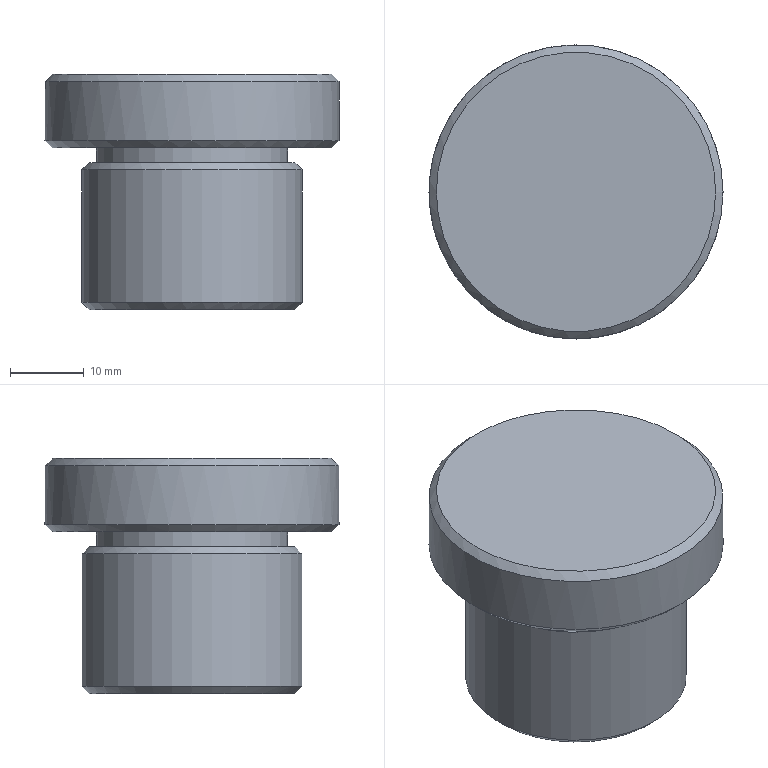Component | NX | DOWEL_PIN | 1 solid | 11 faces | box 40 x 40 x 32 mm | volume 27550 mm3 | plane 4 | cone 4 | cylinder 3 | commonest cylinder face diameters 30 x1 26 x1 40 x1
STEP:
#1=CARTESIAN_POINT('',(0.,0.,0.));
#2=DIRECTION('',(0.,0.,1.));
#3=DIRECTION('',(1.,0.,0.));
#4=AXIS2_PLACEMENT_3D('',#1,#2,#3);
#5=CARTESIAN_POINT('',(14.,0.,71.));
#6=VERTEX_POINT('',#5);
#7=CARTESIAN_POINT('',(0.,0.,71.));
#8=DIRECTION('',(0.,0.,1.));
#9=DIRECTION('',(1.,0.,0.));
#10=AXIS2_PLACEMENT_3D('',#7,#8,#9);
#11=CIRCLE('',#10,14.);
#12=CARTESIAN_POINT('',(0.,0.,71.));
#13=DIRECTION('',(0.,0.,1.));
#14=DIRECTION('',(1.,0.,0.));
#15=AXIS2_PLACEMENT_3D('',#12,#13,#14);
#16=PLANE('',#15);
#17=CARTESIAN_POINT('',(0.,0.));
#18=DIRECTION('',(1.,0.));
#19=AXIS2_PLACEMENT_2D('',#17,#18);
#20=CIRCLE('',#19,14.);
#21=(GEOMETRIC_REPRESENTATION_CONTEXT(2)PARAMETRIC_REPRESENTATION_CONTEXT()REPRESENTATION_CONTEXT('',''));
#22=DEFINITIONAL_REPRESENTATION('',(#20),#21);
#23=PCURVE('',#16,#22);
#24=CARTESIAN_POINT('',(0.,0.,70.));
#25=DIRECTION('',(0.,0.,-1.));
#26=DIRECTION('',(-1.,0.,0.));
#27=AXIS2_PLACEMENT_3D('',#24,#25,#26);
#28=CONICAL_SURFACE('',#27,15.,0.7854);
#29=CARTESIAN_POINT('',(9.425,-1.));
#30=DIRECTION('',(-1.,0.));
#31=VECTOR('',#30,1.);
#32=LINE('',#29,#31);
#33=(GEOMETRIC_REPRESENTATION_CONTEXT(2)PARAMETRIC_REPRESENTATION_CONTEXT()REPRESENTATION_CONTEXT('',''));
#34=DEFINITIONAL_REPRESENTATION('',(#32),#33);
#35=PCURVE('',#28,#34);
#36=SURFACE_CURVE('',#11,(#23,#35),.PCURVE_S1.);
#37=EDGE_CURVE('',#6,#6,#36,.T.);
#38=ORIENTED_EDGE('',*,*,#37,.T.);
#39=EDGE_LOOP('',(#38));
#40=FACE_BOUND('',#39,.T.);
#41=CARTESIAN_POINT('',(13.,0.,71.));
#42=VERTEX_POINT('',#41);
#43=CARTESIAN_POINT('',(0.,0.,71.));
#44=DIRECTION('',(0.,0.,1.));
#45=DIRECTION('',(1.,0.,0.));
#46=AXIS2_PLACEMENT_3D('',#43,#44,#45);
#47=CIRCLE('',#46,13.);
#48=CARTESIAN_POINT('',(0.,0.));
#49=DIRECTION('',(1.,0.));
#50=AXIS2_PLACEMENT_2D('',#48,#49);
#51=CIRCLE('',#50,13.);
#52=(GEOMETRIC_REPRESENTATION_CONTEXT(2)PARAMETRIC_REPRESENTATION_CONTEXT()REPRESENTATION_CONTEXT('',''));
#53=DEFINITIONAL_REPRESENTATION('',(#51),#52);
#54=PCURVE('',#16,#53);
#55=CARTESIAN_POINT('',(0.,0.,71.));
#56=DIRECTION('',(0.,0.,1.));
#57=DIRECTION('',(1.,0.,0.));
#58=AXIS2_PLACEMENT_3D('',#55,#56,#57);
#59=CYLINDRICAL_SURFACE('',#58,13.);
#60=CARTESIAN_POINT('',(0.,0.));
#61=DIRECTION('',(1.,0.));
#62=VECTOR('',#61,1.);
#63=LINE('',#60,#62);
#64=(GEOMETRIC_REPRESENTATION_CONTEXT(2)PARAMETRIC_REPRESENTATION_CONTEXT()REPRESENTATION_CONTEXT('',''));
#65=DEFINITIONAL_REPRESENTATION('',(#63),#64);
#66=PCURVE('',#59,#65);
#67=SURFACE_CURVE('',#47,(#54,#66),.PCURVE_S1.);
#68=EDGE_CURVE('',#42,#42,#67,.T.);
#69=ORIENTED_EDGE('',*,*,#68,.F.);
#70=EDGE_LOOP('',(#69));
#71=FACE_BOUND('',#70,.T.);
#72=ADVANCED_FACE('',(#40,#71),#16,.T.);
#73=CARTESIAN_POINT('',(-14.,0.,51.));
#74=VERTEX_POINT('',#73);
#75=CARTESIAN_POINT('',(0.,0.,51.));
#76=DIRECTION('',(0.,0.,-1.));
#77=DIRECTION('',(-1.,0.,0.));
#78=AXIS2_PLACEMENT_3D('',#75,#76,#77);
#79=CIRCLE('',#78,14.);
#80=CARTESIAN_POINT('',(0.,0.,51.));
#81=DIRECTION('',(0.,0.,-1.));
#82=DIRECTION('',(-1.,0.,0.));
#83=AXIS2_PLACEMENT_3D('',#80,#81,#82);
#84=PLANE('',#83);
#85=CARTESIAN_POINT('',(0.,0.));
#86=DIRECTION('',(1.,0.));
#87=AXIS2_PLACEMENT_2D('',#85,#86);
#88=CIRCLE('',#87,14.);
#89=(GEOMETRIC_REPRESENTATION_CONTEXT(2)PARAMETRIC_REPRESENTATION_CONTEXT()REPRESENTATION_CONTEXT('',''));
#90=DEFINITIONAL_REPRESENTATION('',(#88),#89);
#91=PCURVE('',#84,#90);
#92=CARTESIAN_POINT('',(0.,0.,52.));
#93=DIRECTION('',(0.,0.,1.));
#94=DIRECTION('',(1.,0.,0.));
#95=AXIS2_PLACEMENT_3D('',#92,#93,#94);
#96=CONICAL_SURFACE('',#95,15.,0.7854);
#97=CARTESIAN_POINT('',(9.425,-1.));
#98=DIRECTION('',(-1.,0.));
#99=VECTOR('',#98,1.);
#100=LINE('',#97,#99);
#101=(GEOMETRIC_REPRESENTATION_CONTEXT(2)PARAMETRIC_REPRESENTATION_CONTEXT()REPRESENTATION_CONTEXT('',''));
#102=DEFINITIONAL_REPRESENTATION('',(#100),#101);
#103=PCURVE('',#96,#102);
#104=SURFACE_CURVE('',#79,(#91,#103),.PCURVE_S1.);
#105=EDGE_CURVE('',#74,#74,#104,.T.);
#106=ORIENTED_EDGE('',*,*,#105,.T.);
#107=EDGE_LOOP('',(#106));
#108=FACE_BOUND('',#107,.T.);
#109=ADVANCED_FACE('',(#108),#84,.T.);
#110=CARTESIAN_POINT('',(-15.,0.,52.));
#111=VERTEX_POINT('',#110);
#112=CARTESIAN_POINT('',(15.,-0.,52.));
#113=VERTEX_POINT('',#112);
#114=CARTESIAN_POINT('',(0.,0.,52.));
#115=DIRECTION('',(0.,0.,1.));
#116=DIRECTION('',(-1.,0.,0.));
#117=AXIS2_PLACEMENT_3D('',#114,#115,#116);
#118=CIRCLE('',#117,15.);
#119=CARTESIAN_POINT('',(0.,0.,51.));
#120=DIRECTION('',(0.,0.,1.));
#121=DIRECTION('',(1.,0.,0.));
#122=AXIS2_PLACEMENT_3D('',#119,#120,#121);
#123=CYLINDRICAL_SURFACE('',#122,15.);
#124=CARTESIAN_POINT('',(3.142,1.));
#125=DIRECTION('',(1.,0.));
#126=VECTOR('',#125,1.);
#127=LINE('',#124,#126);
#128=(GEOMETRIC_REPRESENTATION_CONTEXT(2)PARAMETRIC_REPRESENTATION_CONTEXT()REPRESENTATION_CONTEXT('',''));
#129=DEFINITIONAL_REPRESENTATION('',(#127),#128);
#130=PCURVE('',#123,#129);
#131=CARTESIAN_POINT('',(3.142,0.));
#132=DIRECTION('',(1.,0.));
#133=VECTOR('',#132,1.);
#134=LINE('',#131,#133);
#135=(GEOMETRIC_REPRESENTATION_CONTEXT(2)PARAMETRIC_REPRESENTATION_CONTEXT()REPRESENTATION_CONTEXT('',''));
#136=DEFINITIONAL_REPRESENTATION('',(#134),#135);
#137=PCURVE('',#96,#136);
#138=SURFACE_CURVE('',#118,(#130,#137),.PCURVE_S1.);
#139=EDGE_CURVE('',#111,#113,#138,.T.);
#140=ORIENTED_EDGE('',*,*,#139,.T.);
#141=CARTESIAN_POINT('',(15.,0.,70.));
#142=VERTEX_POINT('',#141);
#143=CARTESIAN_POINT('',(15.,0.,52.));
#144=CARTESIAN_POINT('',(15.,0.,70.));
#145=B_SPLINE_CURVE_WITH_KNOTS('',1,(#143,#144),.UNSPECIFIED.,.F.,.F.,(2,2),(1.,19.),.PIECEWISE_BEZIER_KNOTS.);
#146=CARTESIAN_POINT('',(6.283,0.));
#147=DIRECTION('',(0.,1.));
#148=VECTOR('',#147,1.);
#149=LINE('',#146,#148);
#150=(GEOMETRIC_REPRESENTATION_CONTEXT(2)PARAMETRIC_REPRESENTATION_CONTEXT()REPRESENTATION_CONTEXT('',''));
#151=DEFINITIONAL_REPRESENTATION('',(#149),#150);
#152=PCURVE('',#123,#151);
#153=CARTESIAN_POINT('',(0.,0.));
#154=DIRECTION('',(0.,1.));
#155=VECTOR('',#154,1.);
#156=LINE('',#153,#155);
#157=(GEOMETRIC_REPRESENTATION_CONTEXT(2)PARAMETRIC_REPRESENTATION_CONTEXT()REPRESENTATION_CONTEXT('',''));
#158=DEFINITIONAL_REPRESENTATION('',(#156),#157);
#159=PCURVE('',#123,#158);
#160=SEAM_CURVE('',#145,(#152,#159),.PCURVE_S1.);
#161=EDGE_CURVE('',#113,#142,#160,.T.);
#162=ORIENTED_EDGE('',*,*,#161,.T.);
#163=CARTESIAN_POINT('',(0.,0.,70.));
#164=DIRECTION('',(0.,0.,-1.));
#165=DIRECTION('',(1.,0.,0.));
#166=AXIS2_PLACEMENT_3D('',#163,#164,#165);
#167=CIRCLE('',#166,15.);
#168=CARTESIAN_POINT('',(6.283,19.));
#169=DIRECTION('',(-1.,0.));
#170=VECTOR('',#169,1.);
#171=LINE('',#168,#170);
#172=(GEOMETRIC_REPRESENTATION_CONTEXT(2)PARAMETRIC_REPRESENTATION_CONTEXT()REPRESENTATION_CONTEXT('',''));
#173=DEFINITIONAL_REPRESENTATION('',(#171),#172);
#174=PCURVE('',#123,#173);
#175=CARTESIAN_POINT('',(3.142,0.));
#176=DIRECTION('',(1.,0.));
#177=VECTOR('',#176,1.);
#178=LINE('',#175,#177);
#179=(GEOMETRIC_REPRESENTATION_CONTEXT(2)PARAMETRIC_REPRESENTATION_CONTEXT()REPRESENTATION_CONTEXT('',''));
#180=DEFINITIONAL_REPRESENTATION('',(#178),#179);
#181=PCURVE('',#28,#180);
#182=SURFACE_CURVE('',#167,(#174,#181),.PCURVE_S1.);
#183=EDGE_CURVE('',#142,#142,#182,.T.);
#184=ORIENTED_EDGE('',*,*,#183,.T.);
#185=ORIENTED_EDGE('',*,*,#161,.F.);
#186=CARTESIAN_POINT('',(0.,0.,52.));
#187=DIRECTION('',(0.,0.,1.));
#188=DIRECTION('',(-1.,0.,0.));
#189=AXIS2_PLACEMENT_3D('',#186,#187,#188);
#190=CIRCLE('',#189,15.);
#191=CARTESIAN_POINT('',(-3.142,1.));
#192=DIRECTION('',(1.,0.));
#193=VECTOR('',#192,1.);
#194=LINE('',#191,#193);
#195=(GEOMETRIC_REPRESENTATION_CONTEXT(2)PARAMETRIC_REPRESENTATION_CONTEXT()REPRESENTATION_CONTEXT('',''));
#196=DEFINITIONAL_REPRESENTATION('',(#194),#195);
#197=PCURVE('',#123,#196);
#198=CARTESIAN_POINT('',(3.142,0.));
#199=DIRECTION('',(1.,0.));
#200=VECTOR('',#199,1.);
#201=LINE('',#198,#200);
#202=(GEOMETRIC_REPRESENTATION_CONTEXT(2)PARAMETRIC_REPRESENTATION_CONTEXT()REPRESENTATION_CONTEXT('',''));
#203=DEFINITIONAL_REPRESENTATION('',(#201),#202);
#204=PCURVE('',#96,#203);
#205=SURFACE_CURVE('',#190,(#197,#204),.PCURVE_S1.);
#206=EDGE_CURVE('',#113,#111,#205,.T.);
#207=ORIENTED_EDGE('',*,*,#206,.T.);
#208=EDGE_LOOP('',(#140,#162,#184,#185,#207));
#209=FACE_BOUND('',#208,.T.);
#210=ADVANCED_FACE('',(#209),#123,.T.);
#211=CARTESIAN_POINT('',(13.,0.,73.));
#212=VERTEX_POINT('',#211);
#213=CARTESIAN_POINT('',(-13.,0.,73.));
#214=VERTEX_POINT('',#213);
#215=CARTESIAN_POINT('',(0.,0.,73.));
#216=DIRECTION('',(0.,0.,1.));
#217=DIRECTION('',(-1.,0.,0.));
#218=AXIS2_PLACEMENT_3D('',#215,#216,#217);
#219=CIRCLE('',#218,13.);
#220=CARTESIAN_POINT('',(-3.142,2.));
#221=DIRECTION('',(1.,0.));
#222=VECTOR('',#221,1.);
#223=LINE('',#220,#222);
#224=(GEOMETRIC_REPRESENTATION_CONTEXT(2)PARAMETRIC_REPRESENTATION_CONTEXT()REPRESENTATION_CONTEXT('',''));
#225=DEFINITIONAL_REPRESENTATION('',(#223),#224);
#226=PCURVE('',#59,#225);
#227=CARTESIAN_POINT('',(0.,0.,73.));
#228=DIRECTION('',(0.,0.,-1.));
#229=DIRECTION('',(-1.,0.,0.));
#230=AXIS2_PLACEMENT_3D('',#227,#228,#229);
#231=PLANE('',#230);
#232=CARTESIAN_POINT('',(13.,0.));
#233=CARTESIAN_POINT('',(13.,-22.517));
#234=CARTESIAN_POINT('',(-6.5,-11.258));
#235=CARTESIAN_POINT('',(-26.,-0.));
#236=CARTESIAN_POINT('',(-6.5,11.258));
#237=CARTESIAN_POINT('',(13.,22.517));
#238=CARTESIAN_POINT('',(13.,0.));
#239=(BOUNDED_CURVE()B_SPLINE_CURVE(2,(#232,#233,#234,#235,#236,#237,#238),.UNSPECIFIED.,.T.,.F.)B_SPLINE_CURVE_WITH_KNOTS((1,2,2,2,2,1),(-2.094,0.,2.094,4.189,6.283,8.378),.UNSPECIFIED.)CURVE()GEOMETRIC_REPRESENTATION_ITEM()RATIONAL_B_SPLINE_CURVE((1.,0.5,1.,0.5,1.,0.5,1.))REPRESENTATION_ITEM(''));
#240=(GEOMETRIC_REPRESENTATION_CONTEXT(2)PARAMETRIC_REPRESENTATION_CONTEXT()REPRESENTATION_CONTEXT('',''));
#241=DEFINITIONAL_REPRESENTATION('',(#239),#240);
#242=PCURVE('',#231,#241);
#243=SURFACE_CURVE('',#219,(#226,#242),.PCURVE_S1.);
#244=EDGE_CURVE('',#212,#214,#243,.T.);
#245=ORIENTED_EDGE('',*,*,#244,.F.);
#246=CARTESIAN_POINT('',(13.,-0.,71.));
#247=CARTESIAN_POINT('',(13.,-0.,73.));
#248=B_SPLINE_CURVE_WITH_KNOTS('',1,(#246,#247),.UNSPECIFIED.,.F.,.F.,(2,2),(0.,2.),.PIECEWISE_BEZIER_KNOTS.);
#249=CARTESIAN_POINT('',(0.,0.));
#250=DIRECTION('',(0.,1.));
#251=VECTOR('',#250,1.);
#252=LINE('',#249,#251);
#253=(GEOMETRIC_REPRESENTATION_CONTEXT(2)PARAMETRIC_REPRESENTATION_CONTEXT()REPRESENTATION_CONTEXT('',''));
#254=DEFINITIONAL_REPRESENTATION('',(#252),#253);
#255=PCURVE('',#59,#254);
#256=CARTESIAN_POINT('',(6.283,0.));
#257=DIRECTION('',(0.,1.));
#258=VECTOR('',#257,1.);
#259=LINE('',#256,#258);
#260=(GEOMETRIC_REPRESENTATION_CONTEXT(2)PARAMETRIC_REPRESENTATION_CONTEXT()REPRESENTATION_CONTEXT('',''));
#261=DEFINITIONAL_REPRESENTATION('',(#259),#260);
#262=PCURVE('',#59,#261);
#263=SEAM_CURVE('',#248,(#255,#262),.PCURVE_S1.);
#264=EDGE_CURVE('',#42,#212,#263,.T.);
#265=ORIENTED_EDGE('',*,*,#264,.F.);
#266=ORIENTED_EDGE('',*,*,#68,.T.);
#267=ORIENTED_EDGE('',*,*,#264,.T.);
#268=CARTESIAN_POINT('',(0.,0.,73.));
#269=DIRECTION('',(0.,0.,1.));
#270=DIRECTION('',(-1.,0.,0.));
#271=AXIS2_PLACEMENT_3D('',#268,#269,#270);
#272=CIRCLE('',#271,13.);
#273=CARTESIAN_POINT('',(3.142,2.));
#274=DIRECTION('',(1.,0.));
#275=VECTOR('',#274,1.);
#276=LINE('',#273,#275);
#277=(GEOMETRIC_REPRESENTATION_CONTEXT(2)PARAMETRIC_REPRESENTATION_CONTEXT()REPRESENTATION_CONTEXT('',''));
#278=DEFINITIONAL_REPRESENTATION('',(#276),#277);
#279=PCURVE('',#59,#278);
#280=CARTESIAN_POINT('',(13.,0.));
#281=CARTESIAN_POINT('',(13.,-22.517));
#282=CARTESIAN_POINT('',(-6.5,-11.258));
#283=CARTESIAN_POINT('',(-26.,-0.));
#284=CARTESIAN_POINT('',(-6.5,11.258));
#285=CARTESIAN_POINT('',(13.,22.517));
#286=CARTESIAN_POINT('',(13.,0.));
#287=(BOUNDED_CURVE()B_SPLINE_CURVE(2,(#280,#281,#282,#283,#284,#285,#286),.UNSPECIFIED.,.T.,.F.)B_SPLINE_CURVE_WITH_KNOTS((1,2,2,2,2,1),(-2.094,0.,2.094,4.189,6.283,8.378),.UNSPECIFIED.)CURVE()GEOMETRIC_REPRESENTATION_ITEM()RATIONAL_B_SPLINE_CURVE((1.,0.5,1.,0.5,1.,0.5,1.))REPRESENTATION_ITEM(''));
#288=(GEOMETRIC_REPRESENTATION_CONTEXT(2)PARAMETRIC_REPRESENTATION_CONTEXT()REPRESENTATION_CONTEXT('',''));
#289=DEFINITIONAL_REPRESENTATION('',(#287),#288);
#290=PCURVE('',#231,#289);
#291=SURFACE_CURVE('',#272,(#279,#290),.PCURVE_S1.);
#292=EDGE_CURVE('',#214,#212,#291,.T.);
#293=ORIENTED_EDGE('',*,*,#292,.F.);
#294=EDGE_LOOP('',(#245,#265,#266,#267,#293));
#295=FACE_BOUND('',#294,.T.);
#296=ADVANCED_FACE('',(#295),#59,.T.);
#297=CARTESIAN_POINT('',(19.,0.,83.));
#298=VERTEX_POINT('',#297);
#299=CARTESIAN_POINT('',(0.,0.,83.));
#300=DIRECTION('',(0.,0.,1.));
#301=DIRECTION('',(1.,0.,0.));
#302=AXIS2_PLACEMENT_3D('',#299,#300,#301);
#303=CIRCLE('',#302,19.);
#304=CARTESIAN_POINT('',(0.,0.,83.));
#305=DIRECTION('',(0.,0.,1.));
#306=DIRECTION('',(1.,0.,0.));
#307=AXIS2_PLACEMENT_3D('',#304,#305,#306);
#308=PLANE('',#307);
#309=CARTESIAN_POINT('',(0.,0.));
#310=DIRECTION('',(1.,0.));
#311=AXIS2_PLACEMENT_2D('',#309,#310);
#312=CIRCLE('',#311,19.);
#313=(GEOMETRIC_REPRESENTATION_CONTEXT(2)PARAMETRIC_REPRESENTATION_CONTEXT()REPRESENTATION_CONTEXT('',''));
#314=DEFINITIONAL_REPRESENTATION('',(#312),#313);
#315=PCURVE('',#308,#314);
#316=CARTESIAN_POINT('',(0.,0.,82.));
#317=DIRECTION('',(0.,0.,-1.));
#318=DIRECTION('',(-1.,0.,0.));
#319=AXIS2_PLACEMENT_3D('',#316,#317,#318);
#320=CONICAL_SURFACE('',#319,20.,0.7854);
#321=CARTESIAN_POINT('',(9.425,-1.));
#322=DIRECTION('',(-1.,0.));
#323=VECTOR('',#322,1.);
#324=LINE('',#321,#323);
#325=(GEOMETRIC_REPRESENTATION_CONTEXT(2)PARAMETRIC_REPRESENTATION_CONTEXT()REPRESENTATION_CONTEXT('',''));
#326=DEFINITIONAL_REPRESENTATION('',(#324),#325);
#327=PCURVE('',#320,#326);
#328=SURFACE_CURVE('',#303,(#315,#327),.PCURVE_S1.);
#329=EDGE_CURVE('',#298,#298,#328,.T.);
#330=ORIENTED_EDGE('',*,*,#329,.T.);
#331=EDGE_LOOP('',(#330));
#332=FACE_BOUND('',#331,.T.);
#333=ADVANCED_FACE('',(#332),#308,.T.);
#334=CARTESIAN_POINT('',(-19.,0.,73.));
#335=VERTEX_POINT('',#334);
#336=CARTESIAN_POINT('',(0.,0.,73.));
#337=DIRECTION('',(0.,0.,-1.));
#338=DIRECTION('',(-1.,0.,0.));
#339=AXIS2_PLACEMENT_3D('',#336,#337,#338);
#340=CIRCLE('',#339,19.);
#341=CARTESIAN_POINT('',(0.,0.));
#342=DIRECTION('',(1.,0.));
#343=AXIS2_PLACEMENT_2D('',#341,#342);
#344=CIRCLE('',#343,19.);
#345=(GEOMETRIC_REPRESENTATION_CONTEXT(2)PARAMETRIC_REPRESENTATION_CONTEXT()REPRESENTATION_CONTEXT('',''));
#346=DEFINITIONAL_REPRESENTATION('',(#344),#345);
#347=PCURVE('',#231,#346);
#348=CARTESIAN_POINT('',(0.,0.,74.));
#349=DIRECTION('',(0.,0.,1.));
#350=DIRECTION('',(1.,0.,0.));
#351=AXIS2_PLACEMENT_3D('',#348,#349,#350);
#352=CONICAL_SURFACE('',#351,20.,0.7854);
#353=CARTESIAN_POINT('',(9.425,-1.));
#354=DIRECTION('',(-1.,0.));
#355=VECTOR('',#354,1.);
#356=LINE('',#353,#355);
#357=(GEOMETRIC_REPRESENTATION_CONTEXT(2)PARAMETRIC_REPRESENTATION_CONTEXT()REPRESENTATION_CONTEXT('',''));
#358=DEFINITIONAL_REPRESENTATION('',(#356),#357);
#359=PCURVE('',#352,#358);
#360=SURFACE_CURVE('',#340,(#347,#359),.PCURVE_S1.);
#361=EDGE_CURVE('',#335,#335,#360,.T.);
#362=ORIENTED_EDGE('',*,*,#361,.T.);
#363=EDGE_LOOP('',(#362));
#364=FACE_BOUND('',#363,.T.);
#365=ORIENTED_EDGE('',*,*,#292,.T.);
#366=ORIENTED_EDGE('',*,*,#244,.T.);
#367=EDGE_LOOP('',(#365,#366));
#368=FACE_BOUND('',#367,.T.);
#369=ADVANCED_FACE('',(#364,#368),#231,.T.);
#370=CARTESIAN_POINT('',(-20.,0.,74.));
#371=VERTEX_POINT('',#370);
#372=CARTESIAN_POINT('',(20.,-0.,74.));
#373=VERTEX_POINT('',#372);
#374=CARTESIAN_POINT('',(0.,0.,74.));
#375=DIRECTION('',(0.,0.,1.));
#376=DIRECTION('',(-1.,0.,0.));
#377=AXIS2_PLACEMENT_3D('',#374,#375,#376);
#378=CIRCLE('',#377,20.);
#379=CARTESIAN_POINT('',(0.,0.,73.));
#380=DIRECTION('',(0.,0.,1.));
#381=DIRECTION('',(1.,0.,0.));
#382=AXIS2_PLACEMENT_3D('',#379,#380,#381);
#383=CYLINDRICAL_SURFACE('',#382,20.);
#384=CARTESIAN_POINT('',(3.142,1.));
#385=DIRECTION('',(1.,0.));
#386=VECTOR('',#385,1.);
#387=LINE('',#384,#386);
#388=(GEOMETRIC_REPRESENTATION_CONTEXT(2)PARAMETRIC_REPRESENTATION_CONTEXT()REPRESENTATION_CONTEXT('',''));
#389=DEFINITIONAL_REPRESENTATION('',(#387),#388);
#390=PCURVE('',#383,#389);
#391=CARTESIAN_POINT('',(3.142,0.));
#392=DIRECTION('',(1.,0.));
#393=VECTOR('',#392,1.);
#394=LINE('',#391,#393);
#395=(GEOMETRIC_REPRESENTATION_CONTEXT(2)PARAMETRIC_REPRESENTATION_CONTEXT()REPRESENTATION_CONTEXT('',''));
#396=DEFINITIONAL_REPRESENTATION('',(#394),#395);
#397=PCURVE('',#352,#396);
#398=SURFACE_CURVE('',#378,(#390,#397),.PCURVE_S1.);
#399=EDGE_CURVE('',#371,#373,#398,.T.);
#400=ORIENTED_EDGE('',*,*,#399,.T.);
#401=CARTESIAN_POINT('',(20.,0.,82.));
#402=VERTEX_POINT('',#401);
#403=CARTESIAN_POINT('',(20.,0.,74.));
#404=CARTESIAN_POINT('',(20.,0.,82.));
#405=B_SPLINE_CURVE_WITH_KNOTS('',1,(#403,#404),.UNSPECIFIED.,.F.,.F.,(2,2),(1.,9.),.PIECEWISE_BEZIER_KNOTS.);
#406=CARTESIAN_POINT('',(6.283,0.));
#407=DIRECTION('',(0.,1.));
#408=VECTOR('',#407,1.);
#409=LINE('',#406,#408);
#410=(GEOMETRIC_REPRESENTATION_CONTEXT(2)PARAMETRIC_REPRESENTATION_CONTEXT()REPRESENTATION_CONTEXT('',''));
#411=DEFINITIONAL_REPRESENTATION('',(#409),#410);
#412=PCURVE('',#383,#411);
#413=CARTESIAN_POINT('',(0.,0.));
#414=DIRECTION('',(0.,1.));
#415=VECTOR('',#414,1.);
#416=LINE('',#413,#415);
#417=(GEOMETRIC_REPRESENTATION_CONTEXT(2)PARAMETRIC_REPRESENTATION_CONTEXT()REPRESENTATION_CONTEXT('',''));
#418=DEFINITIONAL_REPRESENTATION('',(#416),#417);
#419=PCURVE('',#383,#418);
#420=SEAM_CURVE('',#405,(#412,#419),.PCURVE_S1.);
#421=EDGE_CURVE('',#373,#402,#420,.T.);
#422=ORIENTED_EDGE('',*,*,#421,.T.);
#423=CARTESIAN_POINT('',(0.,0.,82.));
#424=DIRECTION('',(0.,0.,-1.));
#425=DIRECTION('',(1.,0.,0.));
#426=AXIS2_PLACEMENT_3D('',#423,#424,#425);
#427=CIRCLE('',#426,20.);
#428=CARTESIAN_POINT('',(6.283,9.));
#429=DIRECTION('',(-1.,0.));
#430=VECTOR('',#429,1.);
#431=LINE('',#428,#430);
#432=(GEOMETRIC_REPRESENTATION_CONTEXT(2)PARAMETRIC_REPRESENTATION_CONTEXT()REPRESENTATION_CONTEXT('',''));
#433=DEFINITIONAL_REPRESENTATION('',(#431),#432);
#434=PCURVE('',#383,#433);
#435=CARTESIAN_POINT('',(3.142,0.));
#436=DIRECTION('',(1.,0.));
#437=VECTOR('',#436,1.);
#438=LINE('',#435,#437);
#439=(GEOMETRIC_REPRESENTATION_CONTEXT(2)PARAMETRIC_REPRESENTATION_CONTEXT()REPRESENTATION_CONTEXT('',''));
#440=DEFINITIONAL_REPRESENTATION('',(#438),#439);
#441=PCURVE('',#320,#440);
#442=SURFACE_CURVE('',#427,(#434,#441),.PCURVE_S1.);
#443=EDGE_CURVE('',#402,#402,#442,.T.);
#444=ORIENTED_EDGE('',*,*,#443,.T.);
#445=ORIENTED_EDGE('',*,*,#421,.F.);
#446=CARTESIAN_POINT('',(0.,0.,74.));
#447=DIRECTION('',(0.,0.,1.));
#448=DIRECTION('',(-1.,0.,0.));
#449=AXIS2_PLACEMENT_3D('',#446,#447,#448);
#450=CIRCLE('',#449,20.);
#451=CARTESIAN_POINT('',(-3.142,1.));
#452=DIRECTION('',(1.,0.));
#453=VECTOR('',#452,1.);
#454=LINE('',#451,#453);
#455=(GEOMETRIC_REPRESENTATION_CONTEXT(2)PARAMETRIC_REPRESENTATION_CONTEXT()REPRESENTATION_CONTEXT('',''));
#456=DEFINITIONAL_REPRESENTATION('',(#454),#455);
#457=PCURVE('',#383,#456);
#458=CARTESIAN_POINT('',(3.142,0.));
#459=DIRECTION('',(1.,0.));
#460=VECTOR('',#459,1.);
#461=LINE('',#458,#460);
#462=(GEOMETRIC_REPRESENTATION_CONTEXT(2)PARAMETRIC_REPRESENTATION_CONTEXT()REPRESENTATION_CONTEXT('',''));
#463=DEFINITIONAL_REPRESENTATION('',(#461),#462);
#464=PCURVE('',#352,#463);
#465=SURFACE_CURVE('',#450,(#457,#464),.PCURVE_S1.);
#466=EDGE_CURVE('',#373,#371,#465,.T.);
#467=ORIENTED_EDGE('',*,*,#466,.T.);
#468=EDGE_LOOP('',(#400,#422,#444,#445,#467));
#469=FACE_BOUND('',#468,.T.);
#470=ADVANCED_FACE('',(#469),#383,.T.);
#471=ORIENTED_EDGE('',*,*,#361,.F.);
#472=CARTESIAN_POINT('',(-19.,0.,73.));
#473=CARTESIAN_POINT('',(-20.,0.,74.));
#474=B_SPLINE_CURVE_WITH_KNOTS('',1,(#472,#473),.UNSPECIFIED.,.F.,.F.,(2,2),(-1.414,0.),.PIECEWISE_BEZIER_KNOTS.);
#475=CARTESIAN_POINT('',(9.425,0.));
#476=DIRECTION('',(0.,1.));
#477=VECTOR('',#476,1.);
#478=LINE('',#475,#477);
#479=(GEOMETRIC_REPRESENTATION_CONTEXT(2)PARAMETRIC_REPRESENTATION_CONTEXT()REPRESENTATION_CONTEXT('',''));
#480=DEFINITIONAL_REPRESENTATION('',(#478),#479);
#481=PCURVE('',#352,#480);
#482=CARTESIAN_POINT('',(3.142,0.));
#483=DIRECTION('',(0.,1.));
#484=VECTOR('',#483,1.);
#485=LINE('',#482,#484);
#486=(GEOMETRIC_REPRESENTATION_CONTEXT(2)PARAMETRIC_REPRESENTATION_CONTEXT()REPRESENTATION_CONTEXT('',''));
#487=DEFINITIONAL_REPRESENTATION('',(#485),#486);
#488=PCURVE('',#352,#487);
#489=SEAM_CURVE('',#474,(#481,#488),.PCURVE_S1.);
#490=EDGE_CURVE('',#335,#371,#489,.T.);
#491=ORIENTED_EDGE('',*,*,#490,.T.);
#492=ORIENTED_EDGE('',*,*,#466,.F.);
#493=ORIENTED_EDGE('',*,*,#399,.F.);
#494=ORIENTED_EDGE('',*,*,#490,.F.);
#495=EDGE_LOOP('',(#471,#491,#492,#493,#494));
#496=FACE_BOUND('',#495,.T.);
#497=ADVANCED_FACE('',(#496),#352,.T.);
#498=ORIENTED_EDGE('',*,*,#329,.F.);
#499=CARTESIAN_POINT('',(19.,0.,83.));
#500=CARTESIAN_POINT('',(20.,0.,82.));
#501=B_SPLINE_CURVE_WITH_KNOTS('',1,(#499,#500),.UNSPECIFIED.,.F.,.F.,(2,2),(-1.414,0.),.PIECEWISE_BEZIER_KNOTS.);
#502=CARTESIAN_POINT('',(9.425,0.));
#503=DIRECTION('',(0.,1.));
#504=VECTOR('',#503,1.);
#505=LINE('',#502,#504);
#506=(GEOMETRIC_REPRESENTATION_CONTEXT(2)PARAMETRIC_REPRESENTATION_CONTEXT()REPRESENTATION_CONTEXT('',''));
#507=DEFINITIONAL_REPRESENTATION('',(#505),#506);
#508=PCURVE('',#320,#507);
#509=CARTESIAN_POINT('',(3.142,0.));
#510=DIRECTION('',(0.,1.));
#511=VECTOR('',#510,1.);
#512=LINE('',#509,#511);
#513=(GEOMETRIC_REPRESENTATION_CONTEXT(2)PARAMETRIC_REPRESENTATION_CONTEXT()REPRESENTATION_CONTEXT('',''));
#514=DEFINITIONAL_REPRESENTATION('',(#512),#513);
#515=PCURVE('',#320,#514);
#516=SEAM_CURVE('',#501,(#508,#515),.PCURVE_S1.);
#517=EDGE_CURVE('',#298,#402,#516,.T.);
#518=ORIENTED_EDGE('',*,*,#517,.T.);
#519=ORIENTED_EDGE('',*,*,#443,.F.);
#520=ORIENTED_EDGE('',*,*,#517,.F.);
#521=EDGE_LOOP('',(#498,#518,#519,#520));
#522=FACE_BOUND('',#521,.T.);
#523=ADVANCED_FACE('',(#522),#320,.T.);
#524=ORIENTED_EDGE('',*,*,#105,.F.);
#525=CARTESIAN_POINT('',(-14.,0.,51.));
#526=CARTESIAN_POINT('',(-15.,0.,52.));
#527=B_SPLINE_CURVE_WITH_KNOTS('',1,(#525,#526),.UNSPECIFIED.,.F.,.F.,(2,2),(-1.414,0.),.PIECEWISE_BEZIER_KNOTS.);
#528=CARTESIAN_POINT('',(9.425,0.));
#529=DIRECTION('',(0.,1.));
#530=VECTOR('',#529,1.);
#531=LINE('',#528,#530);
#532=(GEOMETRIC_REPRESENTATION_CONTEXT(2)PARAMETRIC_REPRESENTATION_CONTEXT()REPRESENTATION_CONTEXT('',''));
#533=DEFINITIONAL_REPRESENTATION('',(#531),#532);
#534=PCURVE('',#96,#533);
#535=CARTESIAN_POINT('',(3.142,0.));
#536=DIRECTION('',(0.,1.));
#537=VECTOR('',#536,1.);
#538=LINE('',#535,#537);
#539=(GEOMETRIC_REPRESENTATION_CONTEXT(2)PARAMETRIC_REPRESENTATION_CONTEXT()REPRESENTATION_CONTEXT('',''));
#540=DEFINITIONAL_REPRESENTATION('',(#538),#539);
#541=PCURVE('',#96,#540);
#542=SEAM_CURVE('',#527,(#534,#541),.PCURVE_S1.);
#543=EDGE_CURVE('',#74,#111,#542,.T.);
#544=ORIENTED_EDGE('',*,*,#543,.T.);
#545=ORIENTED_EDGE('',*,*,#206,.F.);
#546=ORIENTED_EDGE('',*,*,#139,.F.);
#547=ORIENTED_EDGE('',*,*,#543,.F.);
#548=EDGE_LOOP('',(#524,#544,#545,#546,#547));
#549=FACE_BOUND('',#548,.T.);
#550=ADVANCED_FACE('',(#549),#96,.T.);
#551=ORIENTED_EDGE('',*,*,#37,.F.);
#552=CARTESIAN_POINT('',(14.,0.,71.));
#553=CARTESIAN_POINT('',(15.,0.,70.));
#554=B_SPLINE_CURVE_WITH_KNOTS('',1,(#552,#553),.UNSPECIFIED.,.F.,.F.,(2,2),(-1.414,0.),.PIECEWISE_BEZIER_KNOTS.);
#555=CARTESIAN_POINT('',(9.425,0.));
#556=DIRECTION('',(0.,1.));
#557=VECTOR('',#556,1.);
#558=LINE('',#555,#557);
#559=(GEOMETRIC_REPRESENTATION_CONTEXT(2)PARAMETRIC_REPRESENTATION_CONTEXT()REPRESENTATION_CONTEXT('',''));
#560=DEFINITIONAL_REPRESENTATION('',(#558),#559);
#561=PCURVE('',#28,#560);
#562=CARTESIAN_POINT('',(3.142,0.));
#563=DIRECTION('',(0.,1.));
#564=VECTOR('',#563,1.);
#565=LINE('',#562,#564);
#566=(GEOMETRIC_REPRESENTATION_CONTEXT(2)PARAMETRIC_REPRESENTATION_CONTEXT()REPRESENTATION_CONTEXT('',''));
#567=DEFINITIONAL_REPRESENTATION('',(#565),#566);
#568=PCURVE('',#28,#567);
#569=SEAM_CURVE('',#554,(#561,#568),.PCURVE_S1.);
#570=EDGE_CURVE('',#6,#142,#569,.T.);
#571=ORIENTED_EDGE('',*,*,#570,.T.);
#572=ORIENTED_EDGE('',*,*,#183,.F.);
#573=ORIENTED_EDGE('',*,*,#570,.F.);
#574=EDGE_LOOP('',(#551,#571,#572,#573));
#575=FACE_BOUND('',#574,.T.);
#576=ADVANCED_FACE('',(#575),#28,.T.);
#577=CLOSED_SHELL('',(#72,#109,#210,#296,#333,#369,#470,#497,#523,#550,#576));
#578=MANIFOLD_SOLID_BREP('',#577);
#579=(LENGTH_UNIT()NAMED_UNIT(*)SI_UNIT(.MILLI.,.METRE.));
#580=UNCERTAINTY_MEASURE_WITH_UNIT(LENGTH_MEASURE(0.00001),#579,'','');
#581=(NAMED_UNIT(*)PLANE_ANGLE_UNIT()SI_UNIT($,.RADIAN.));
#582=(NAMED_UNIT(*)SI_UNIT($,.STERADIAN.)SOLID_ANGLE_UNIT());
#583=(GEOMETRIC_REPRESENTATION_CONTEXT(3)GLOBAL_UNCERTAINTY_ASSIGNED_CONTEXT((#580))GLOBAL_UNIT_ASSIGNED_CONTEXT((#579,#581,#582))REPRESENTATION_CONTEXT('',''));
#584=ADVANCED_BREP_SHAPE_REPRESENTATION('',(#4,#578),#583);